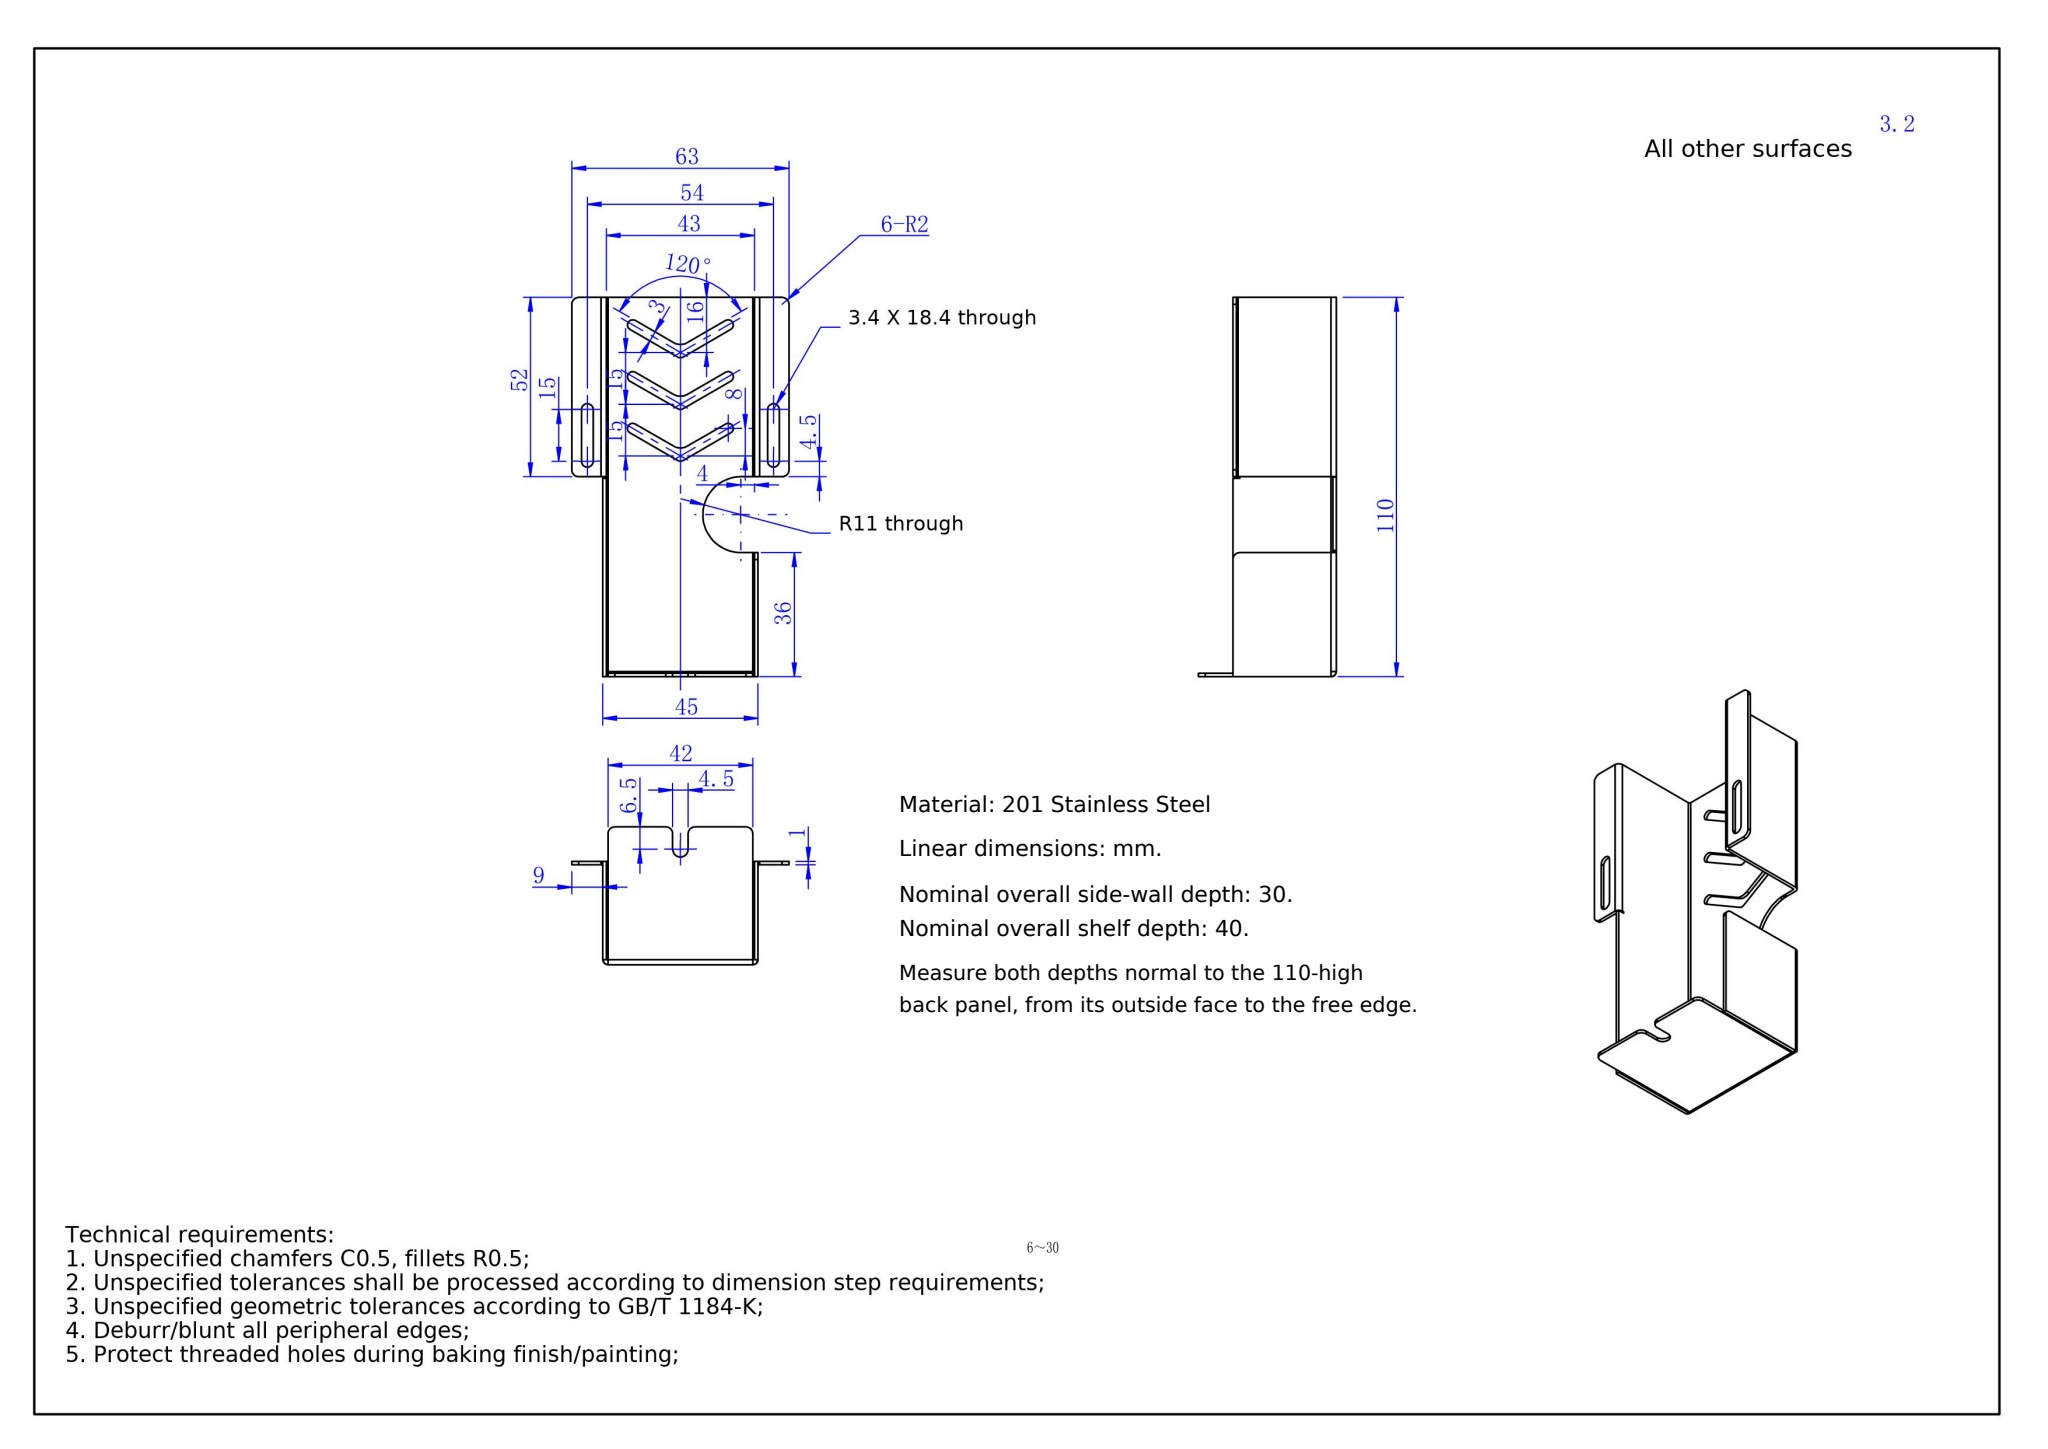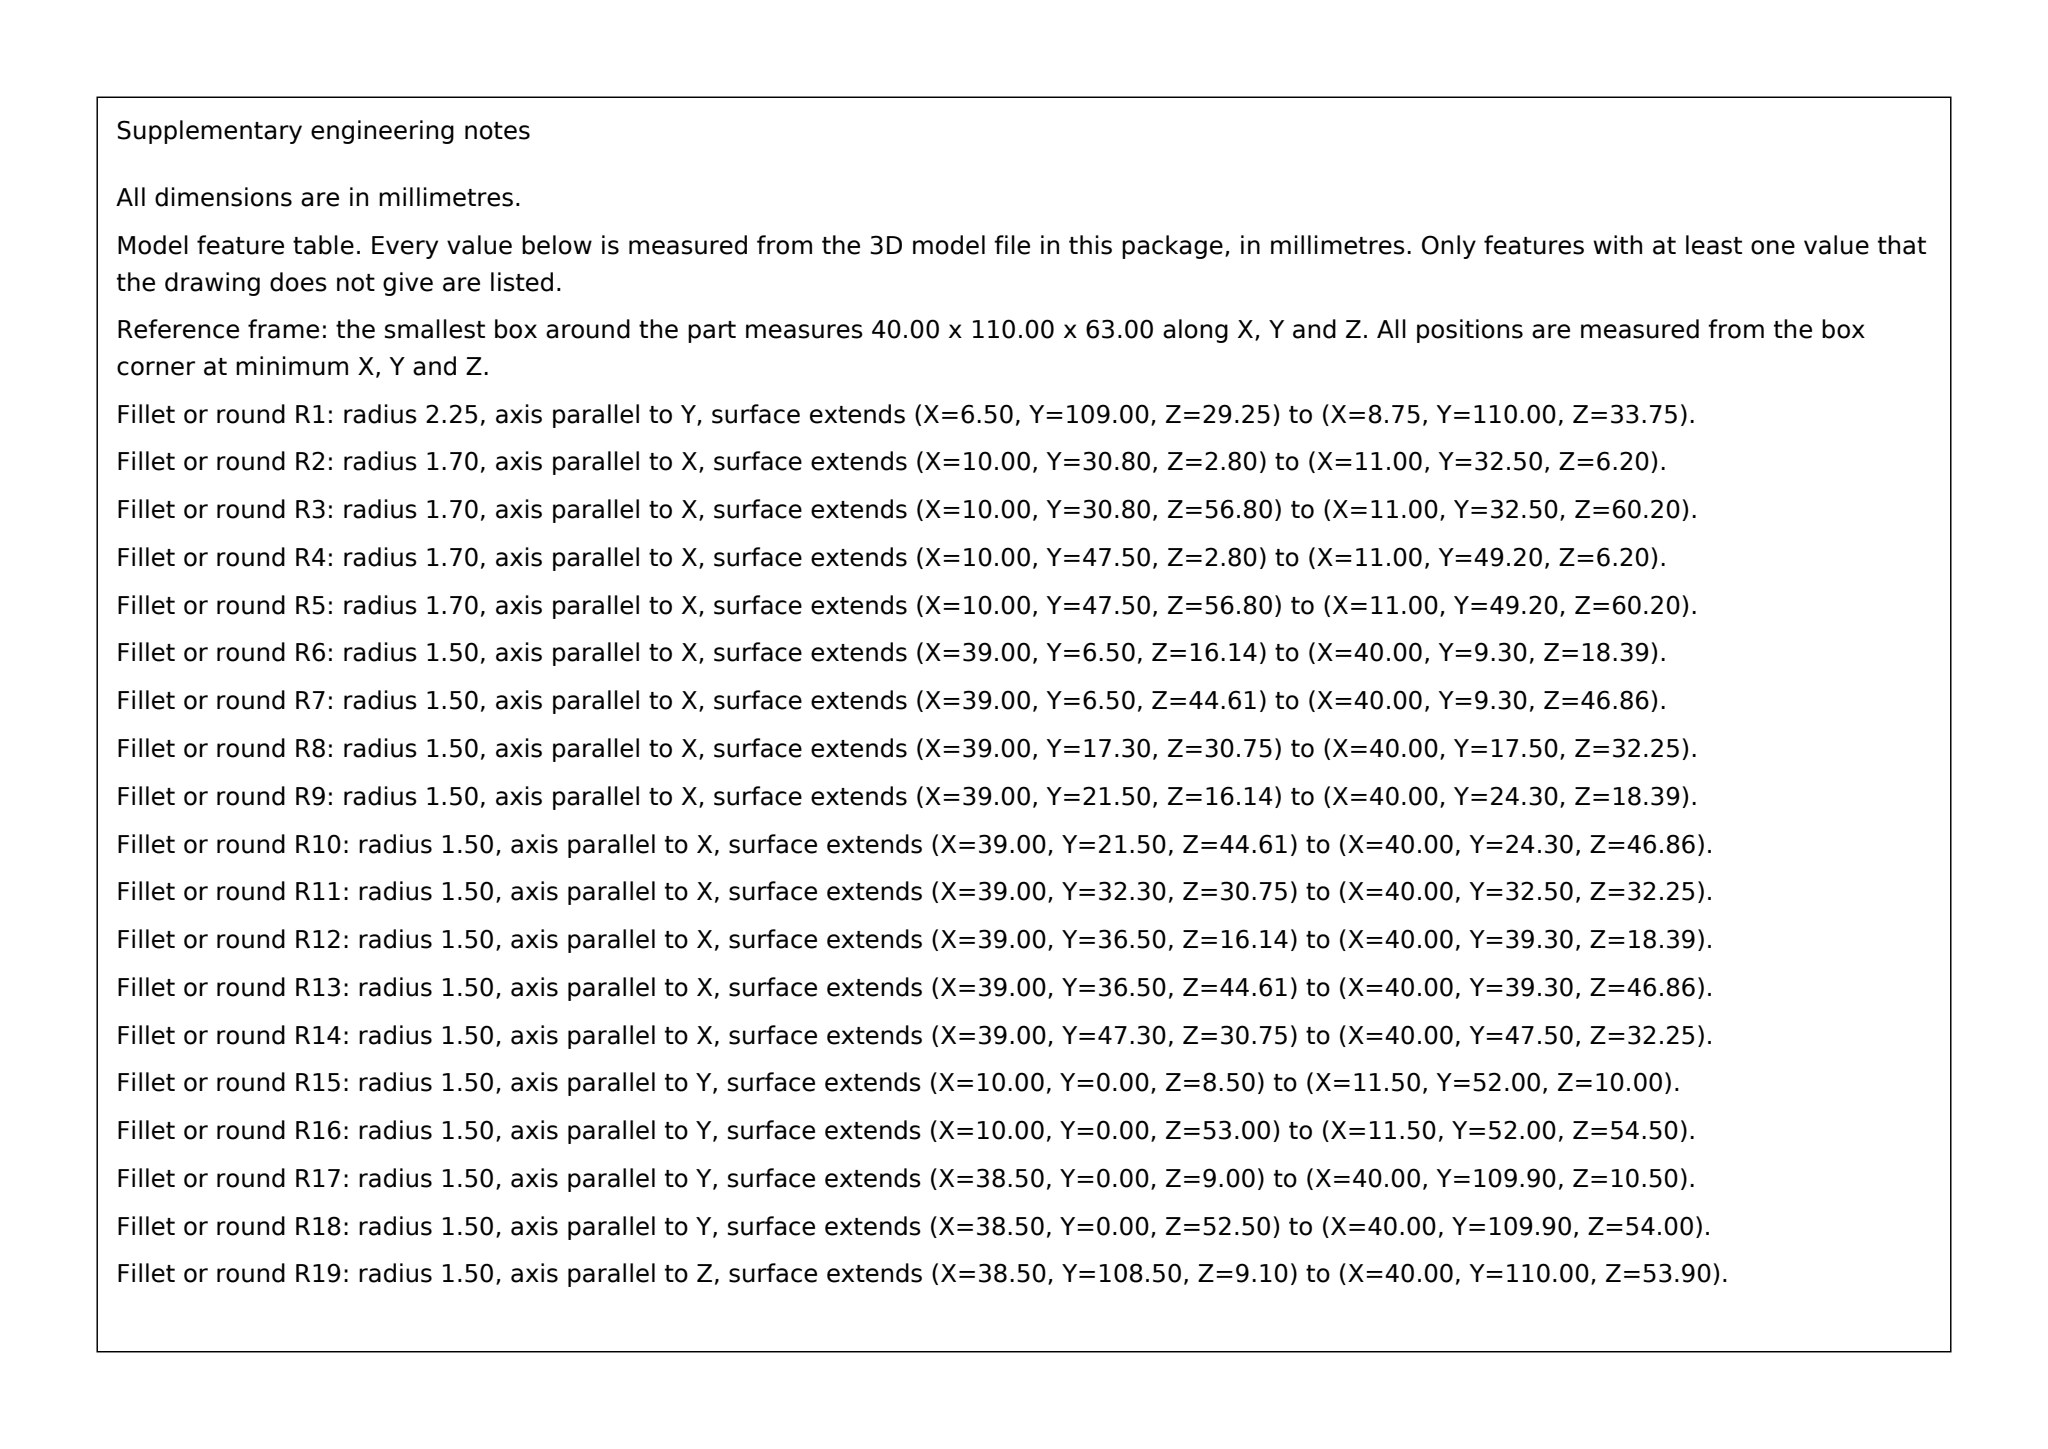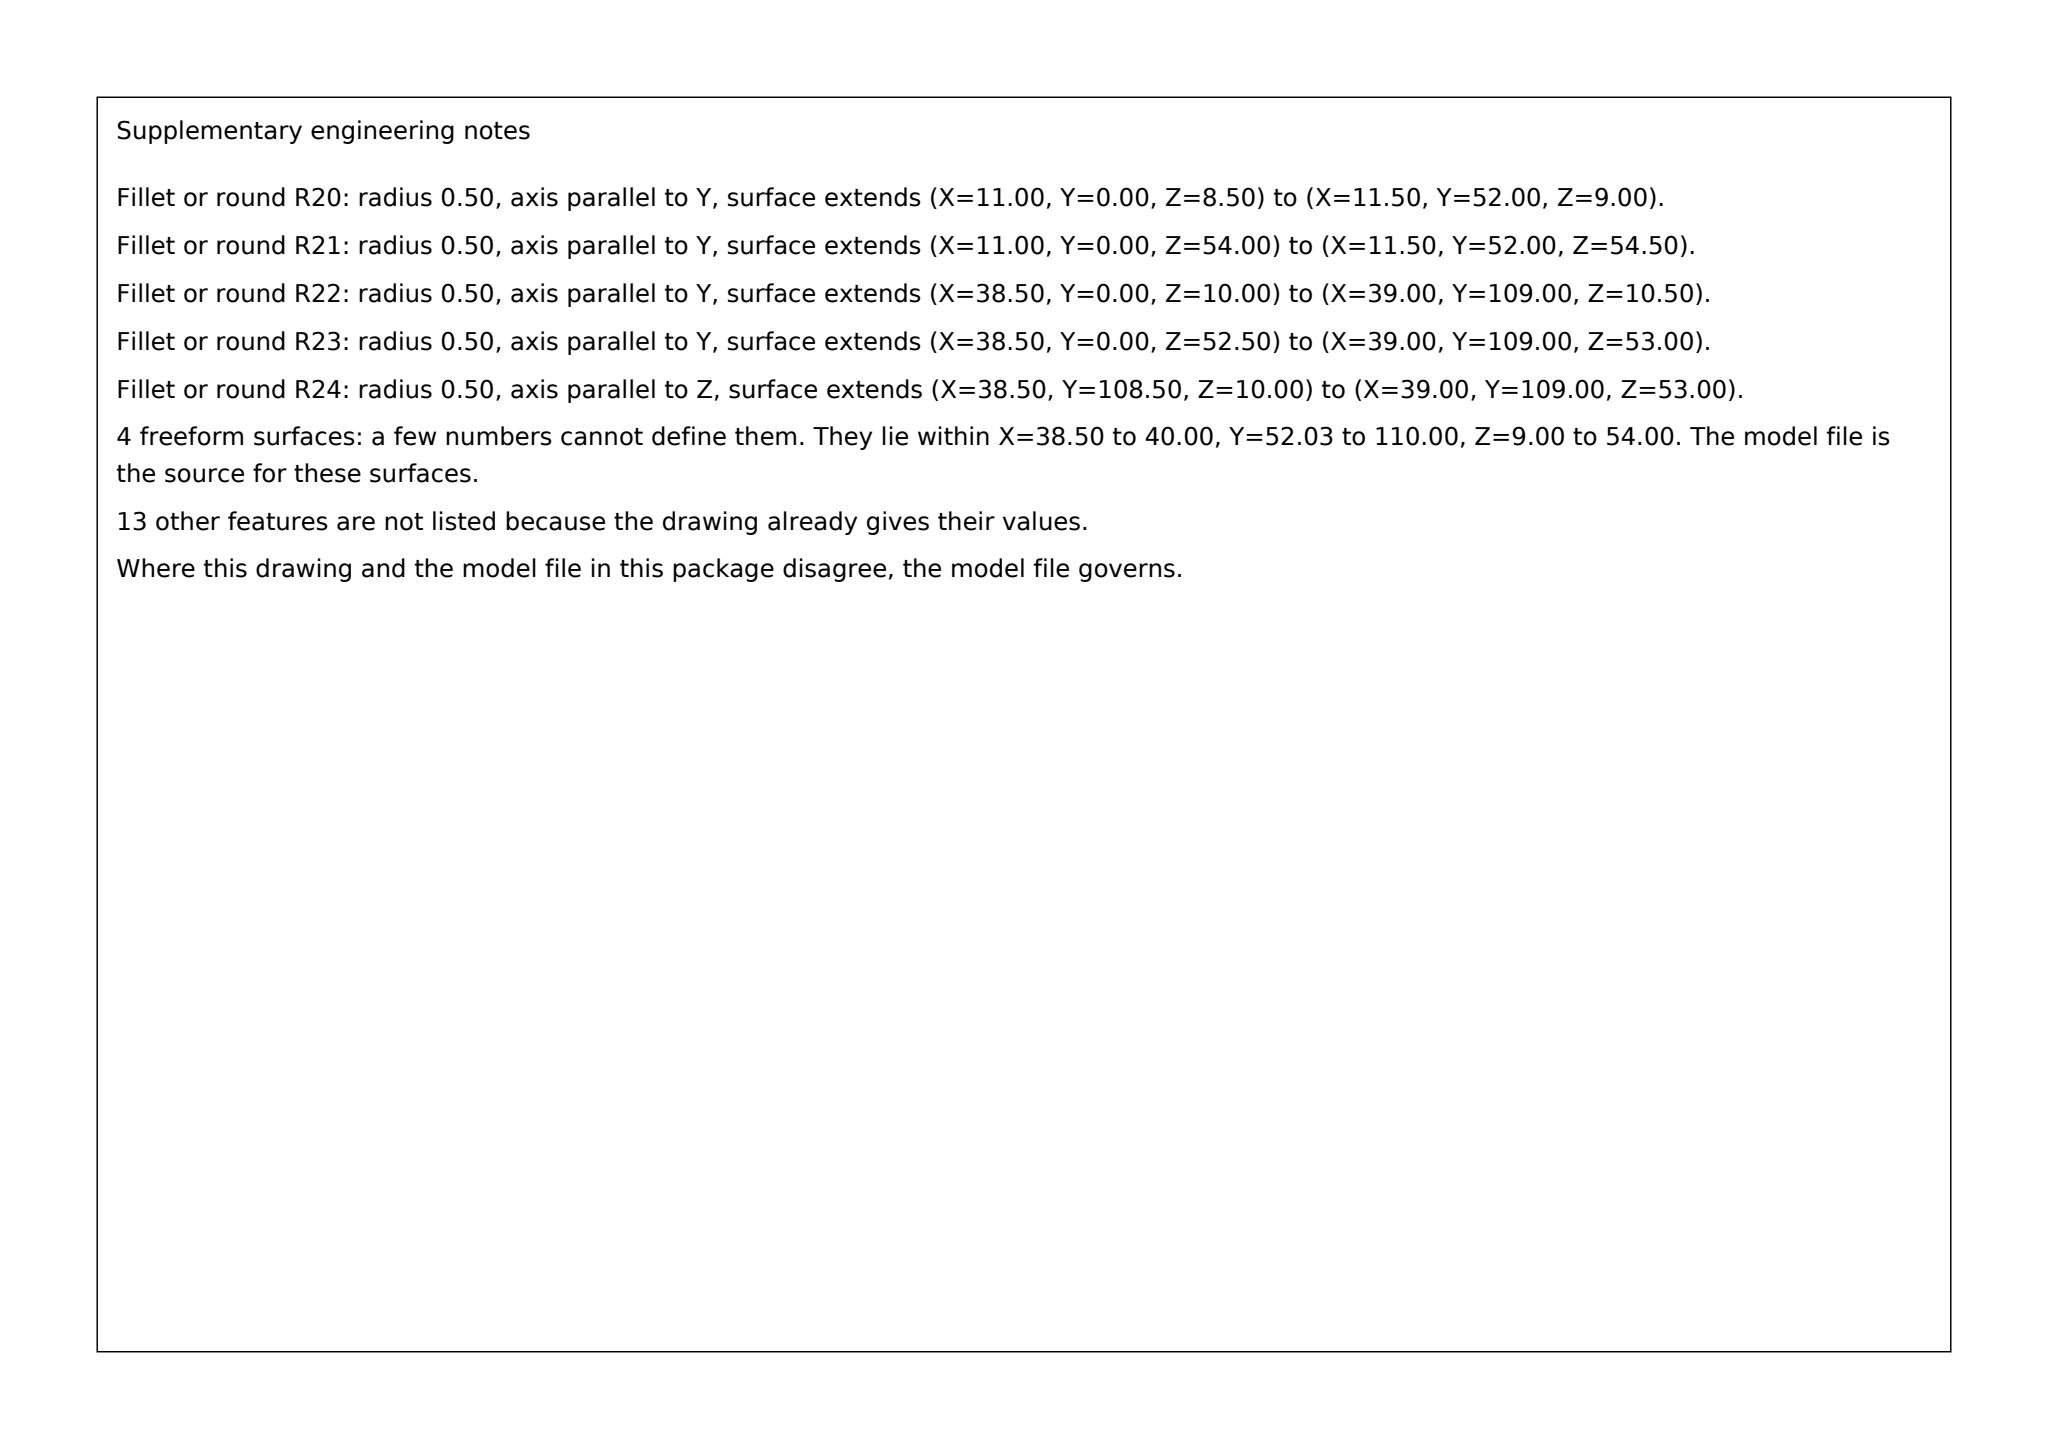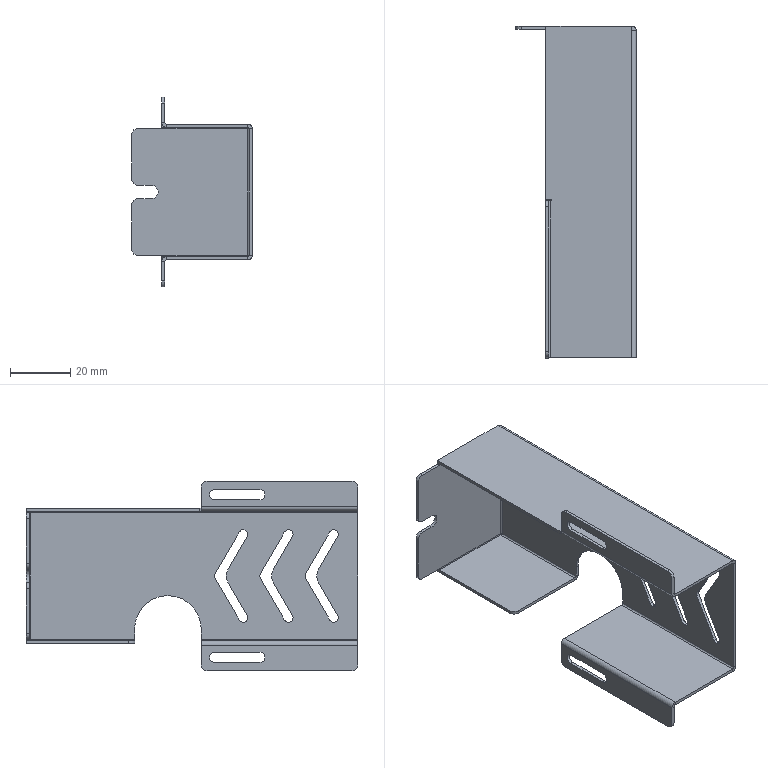Part | SolidWorks | mm | material 201 Stainless Steel | 1 solid | 126 faces | box 40 x 110 x 63 mm | volume 12369 mm3 | plane 70 | cylinder 52 | spline 4 | commonest cylinder face diameters 3 x22 1 x10 4 x9 3.4 x4 8 x3 22 x3 4.5 x1